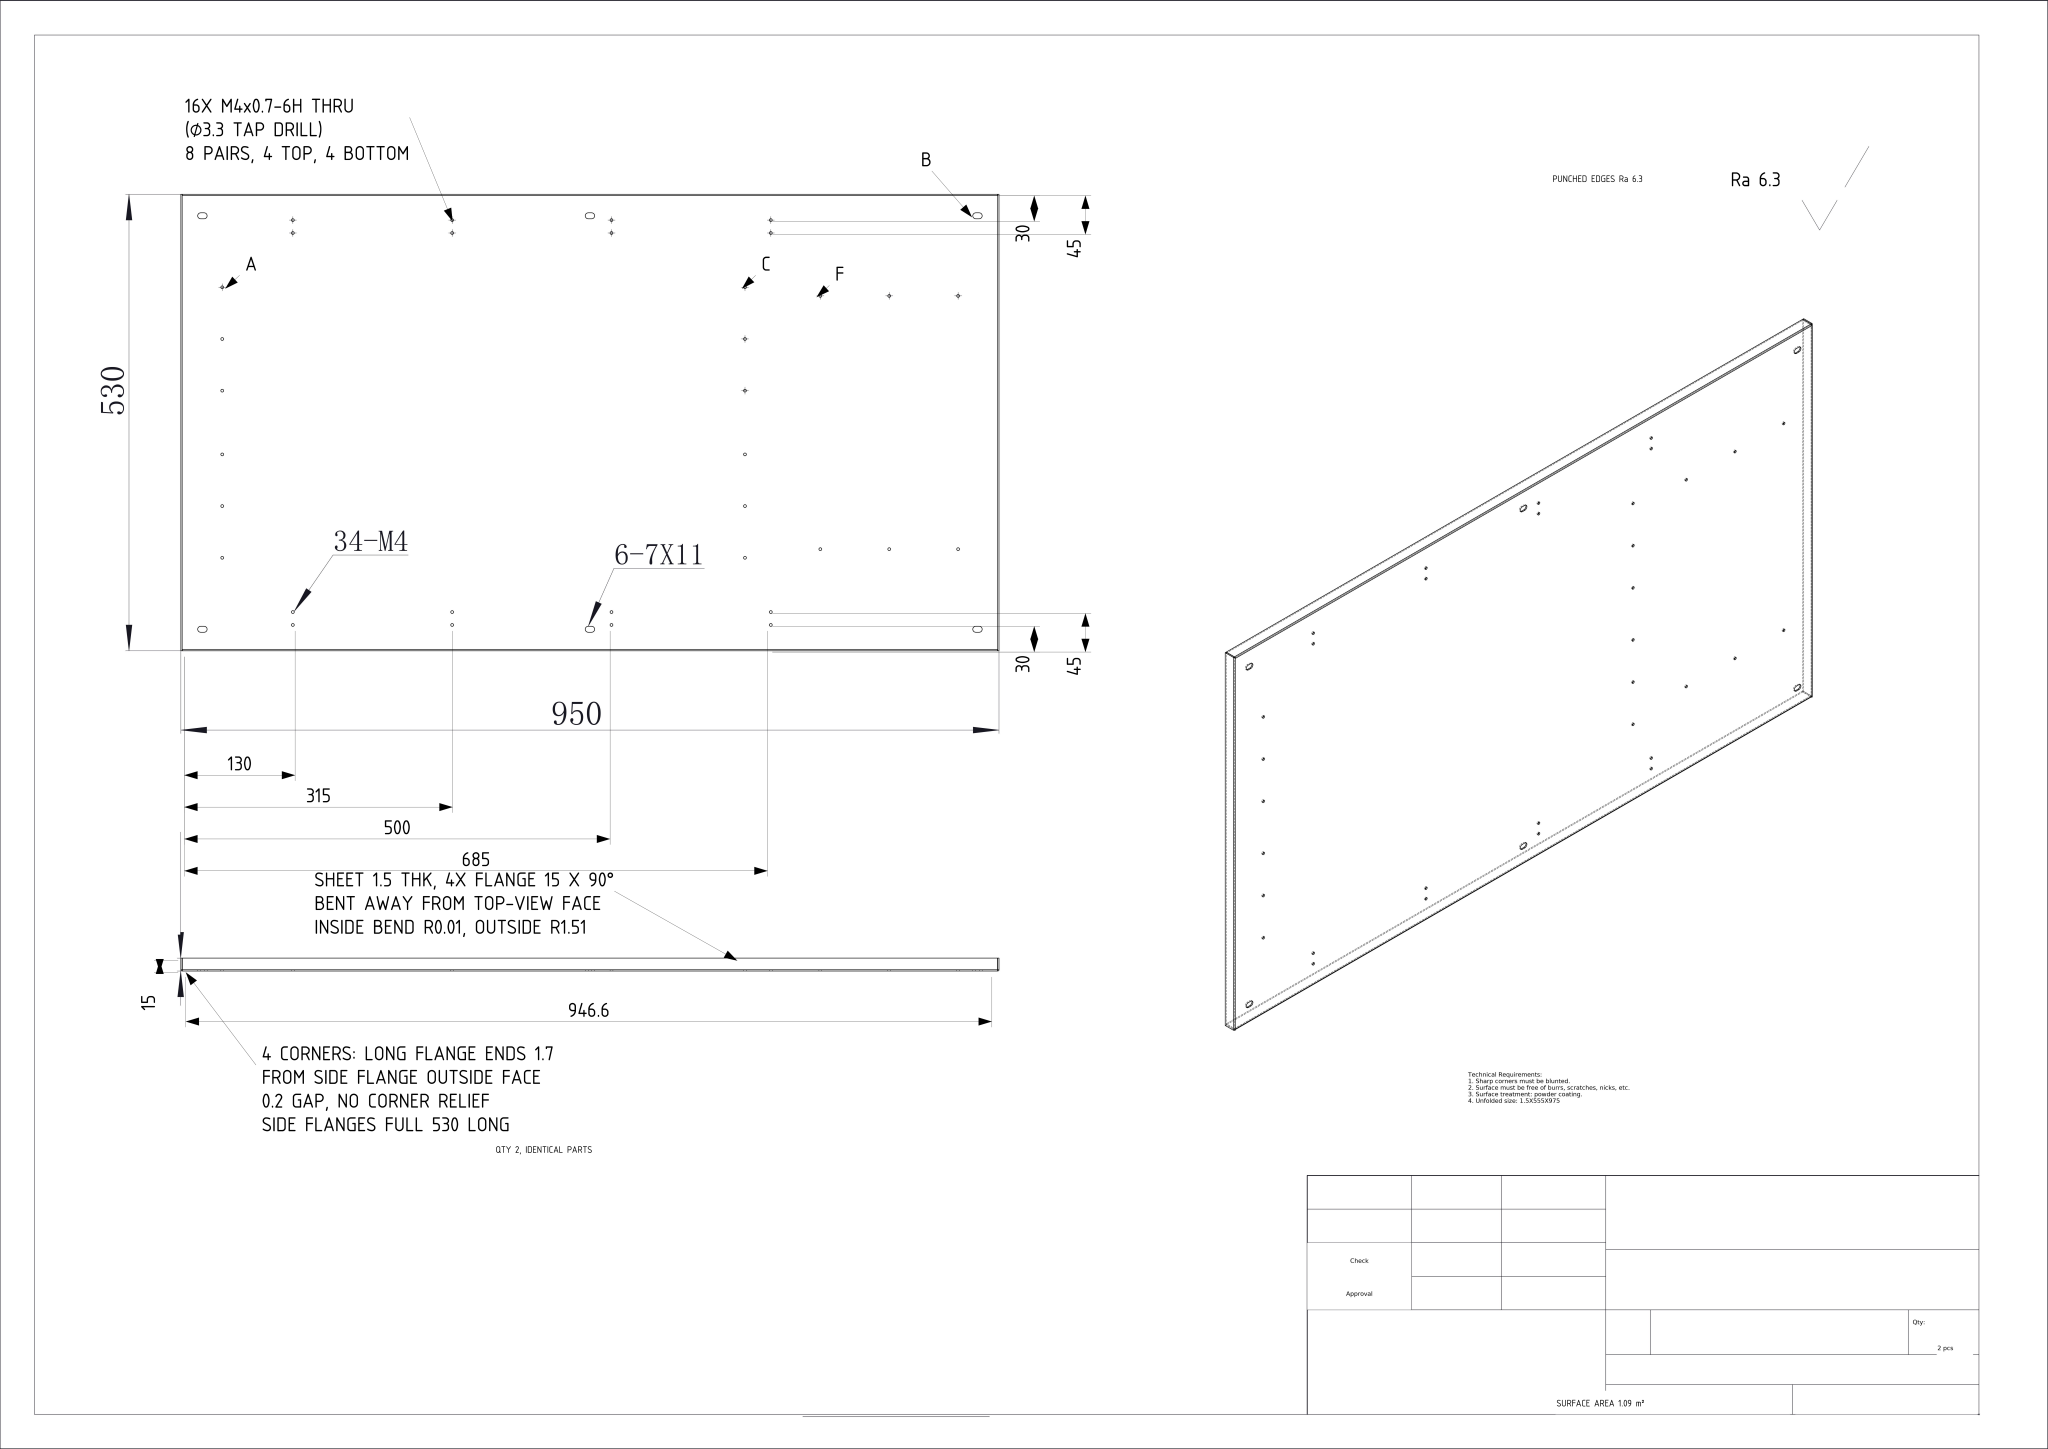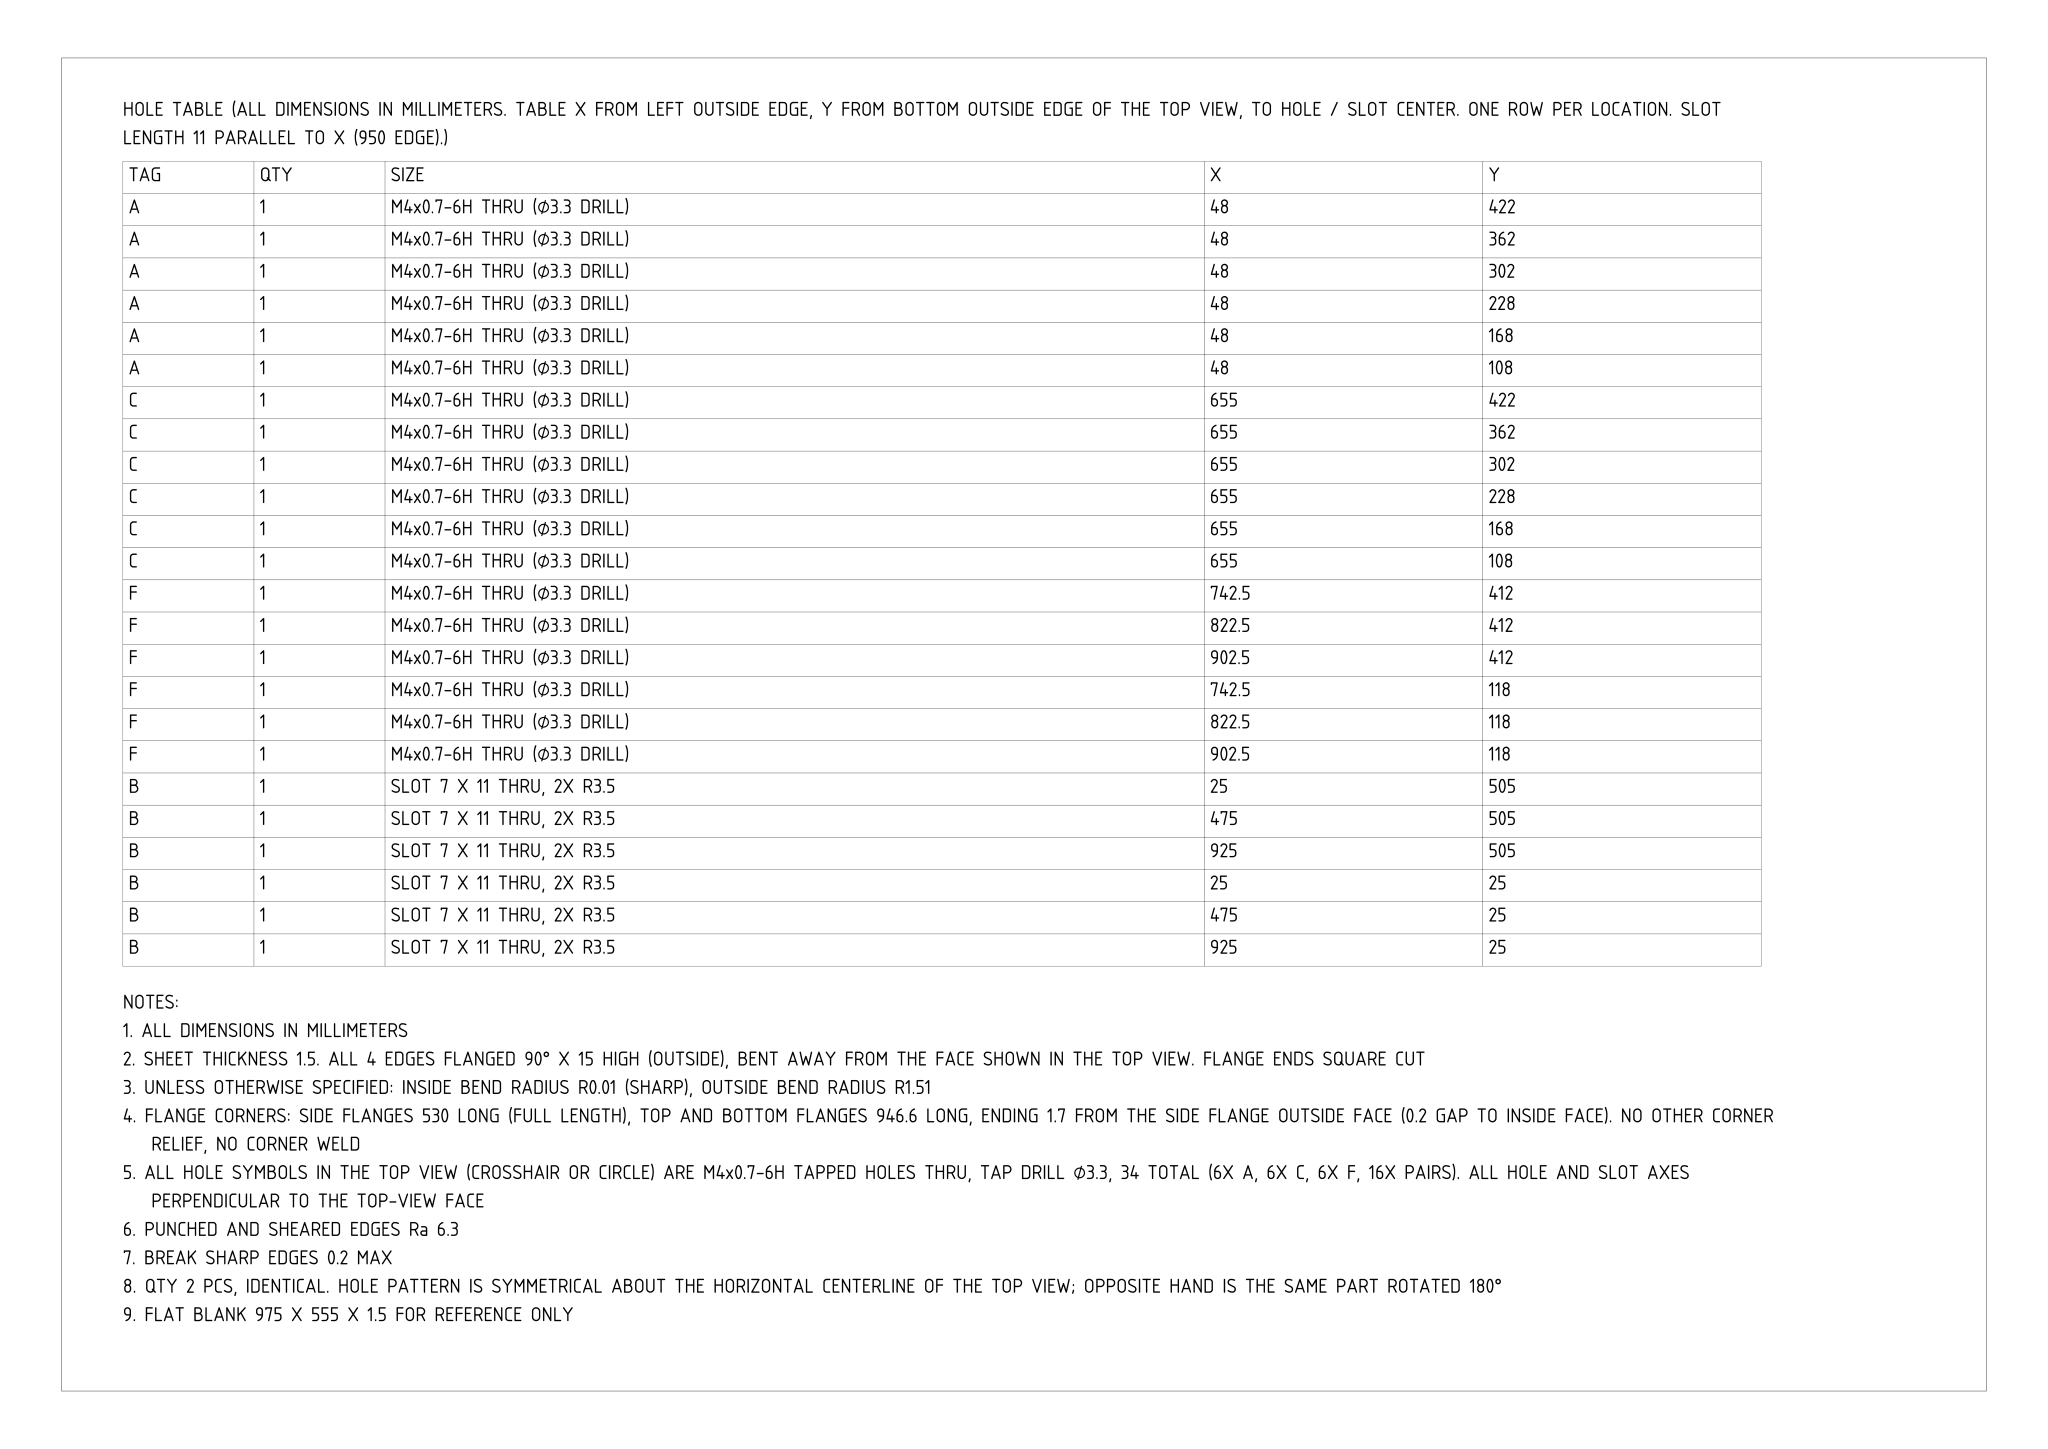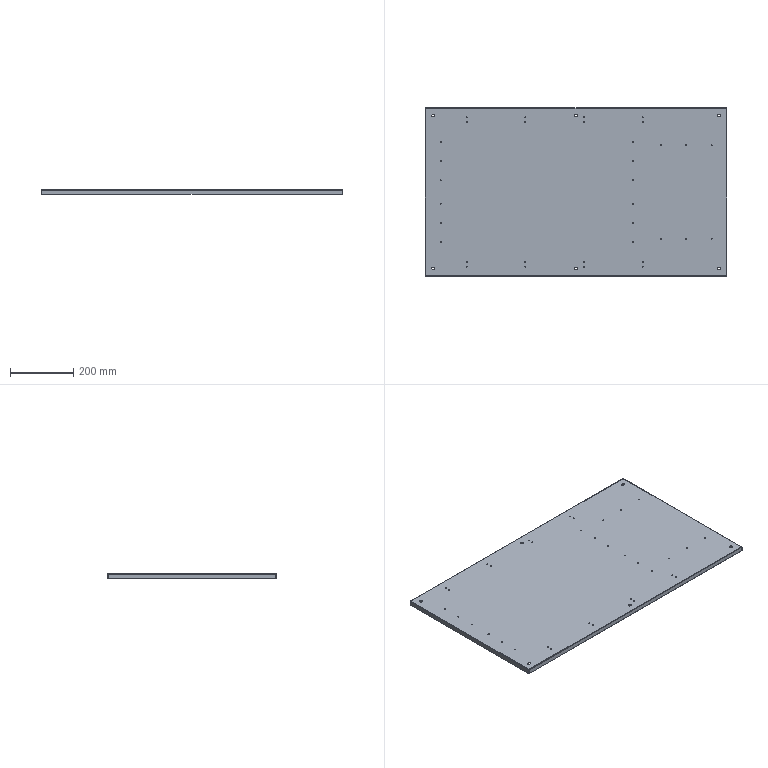Part | NX | mm | 1 solid | 144 faces | box 950 x 530 x 15 mm | volume 812573 mm3 | cylinder 94 | plane 50 | commonest cylinder face diameters 3.3 x68 7 x18 3.02 x4 0.02 x4